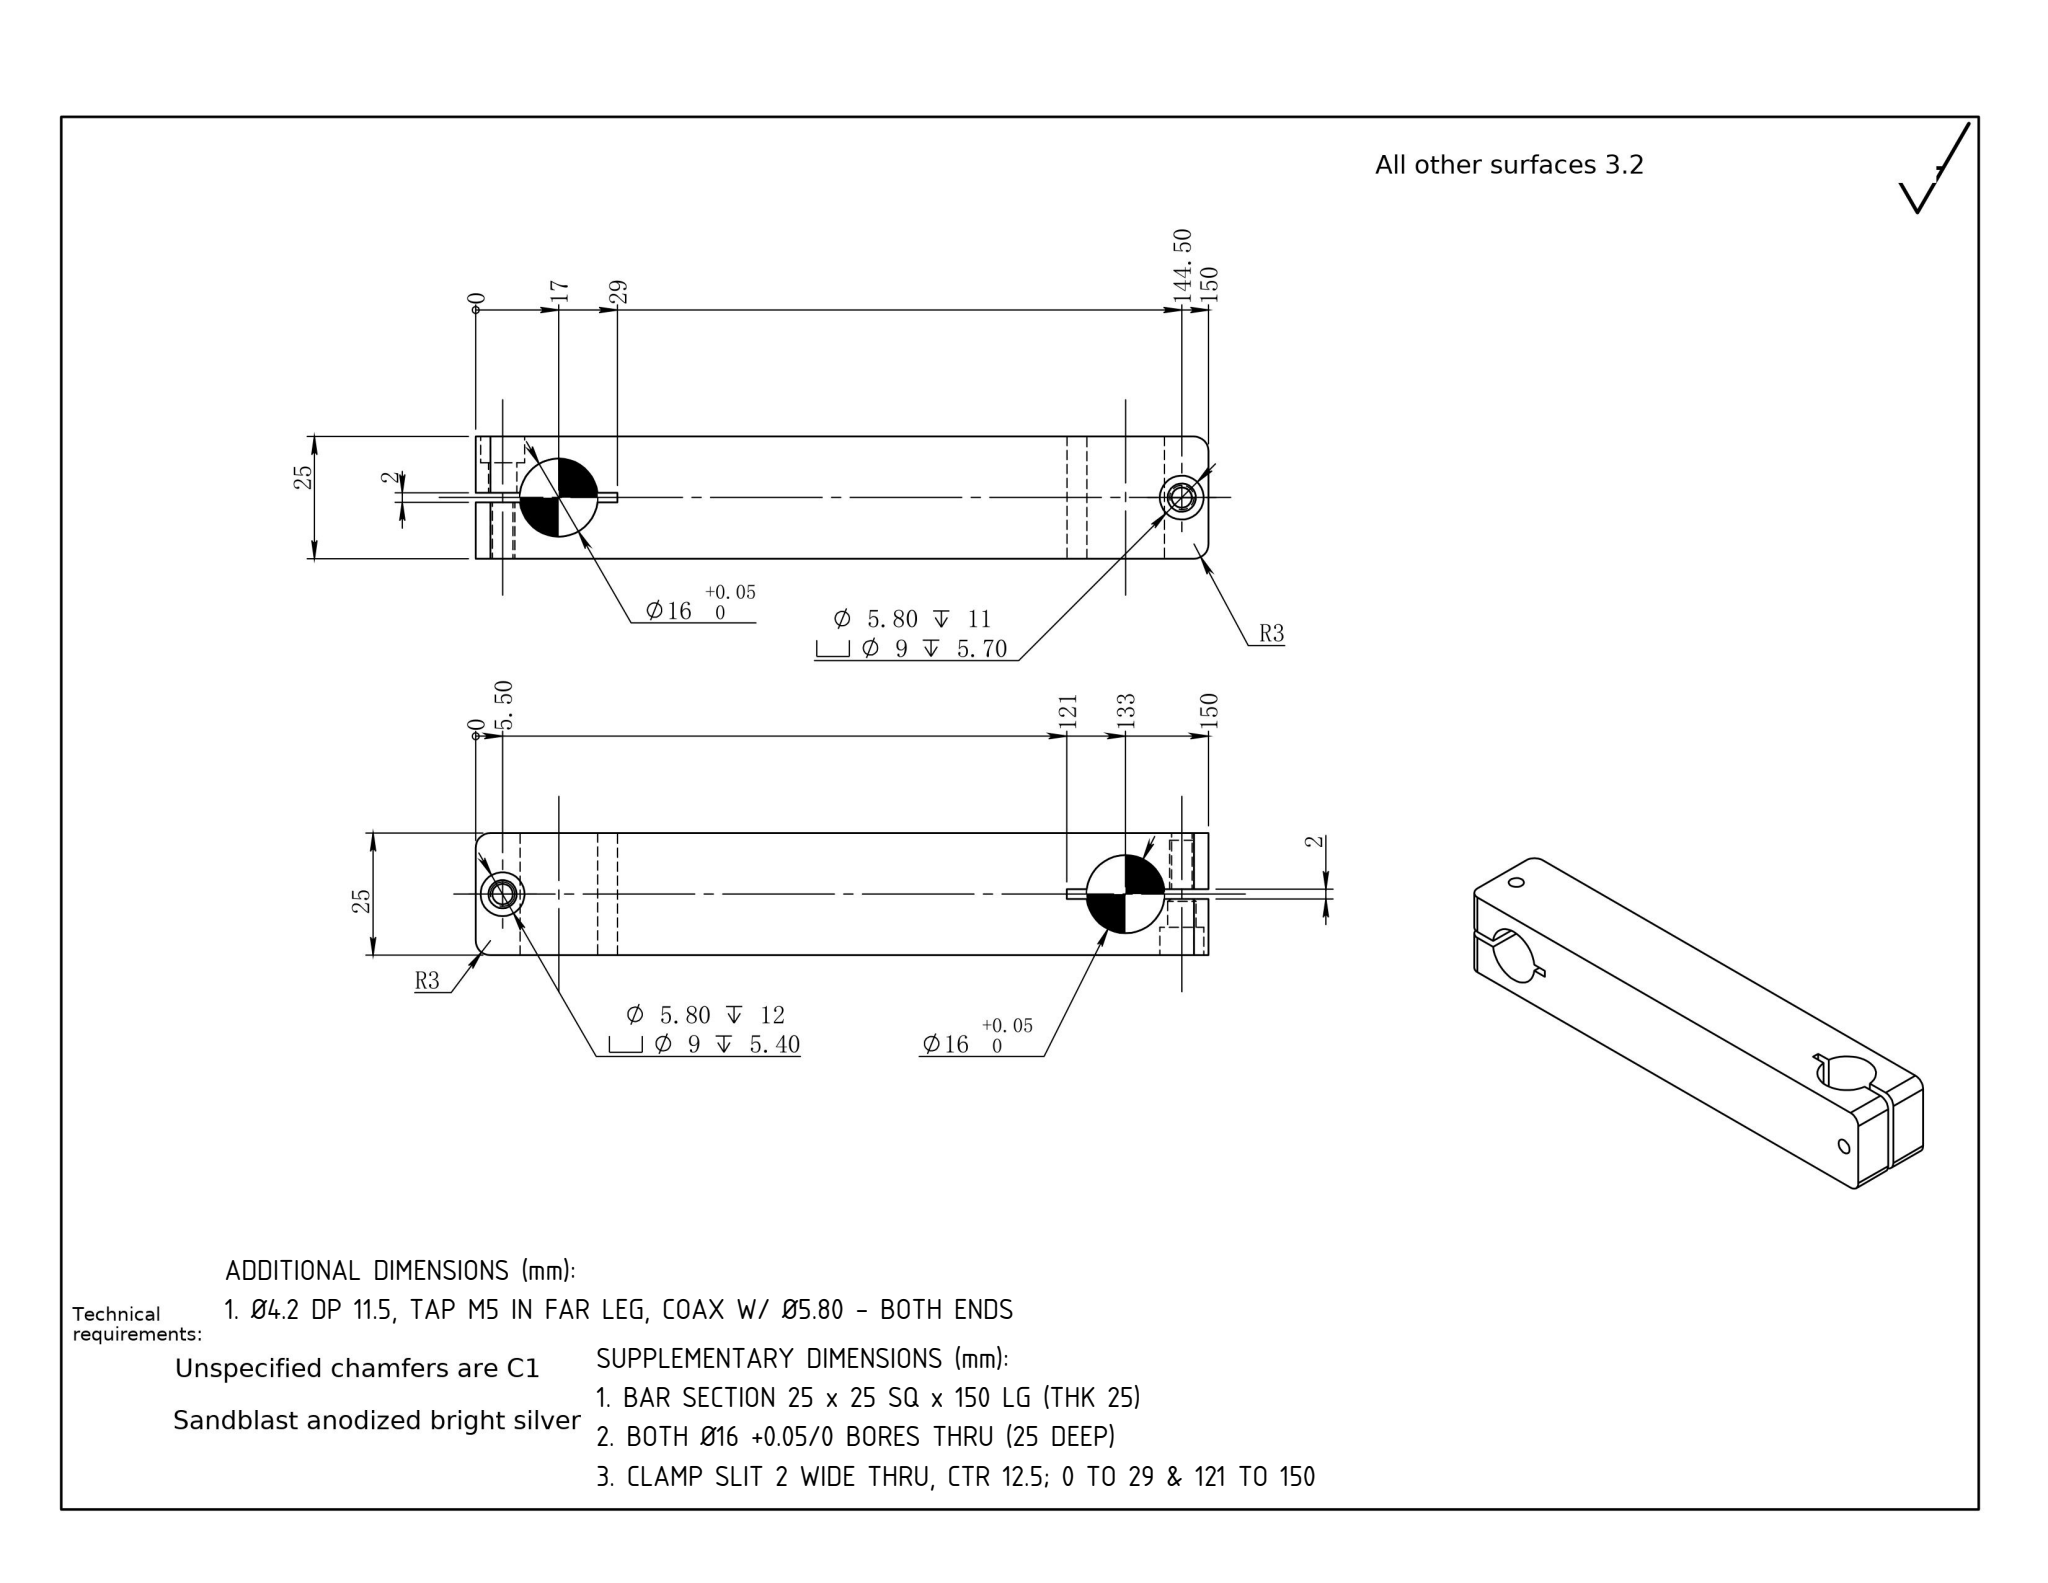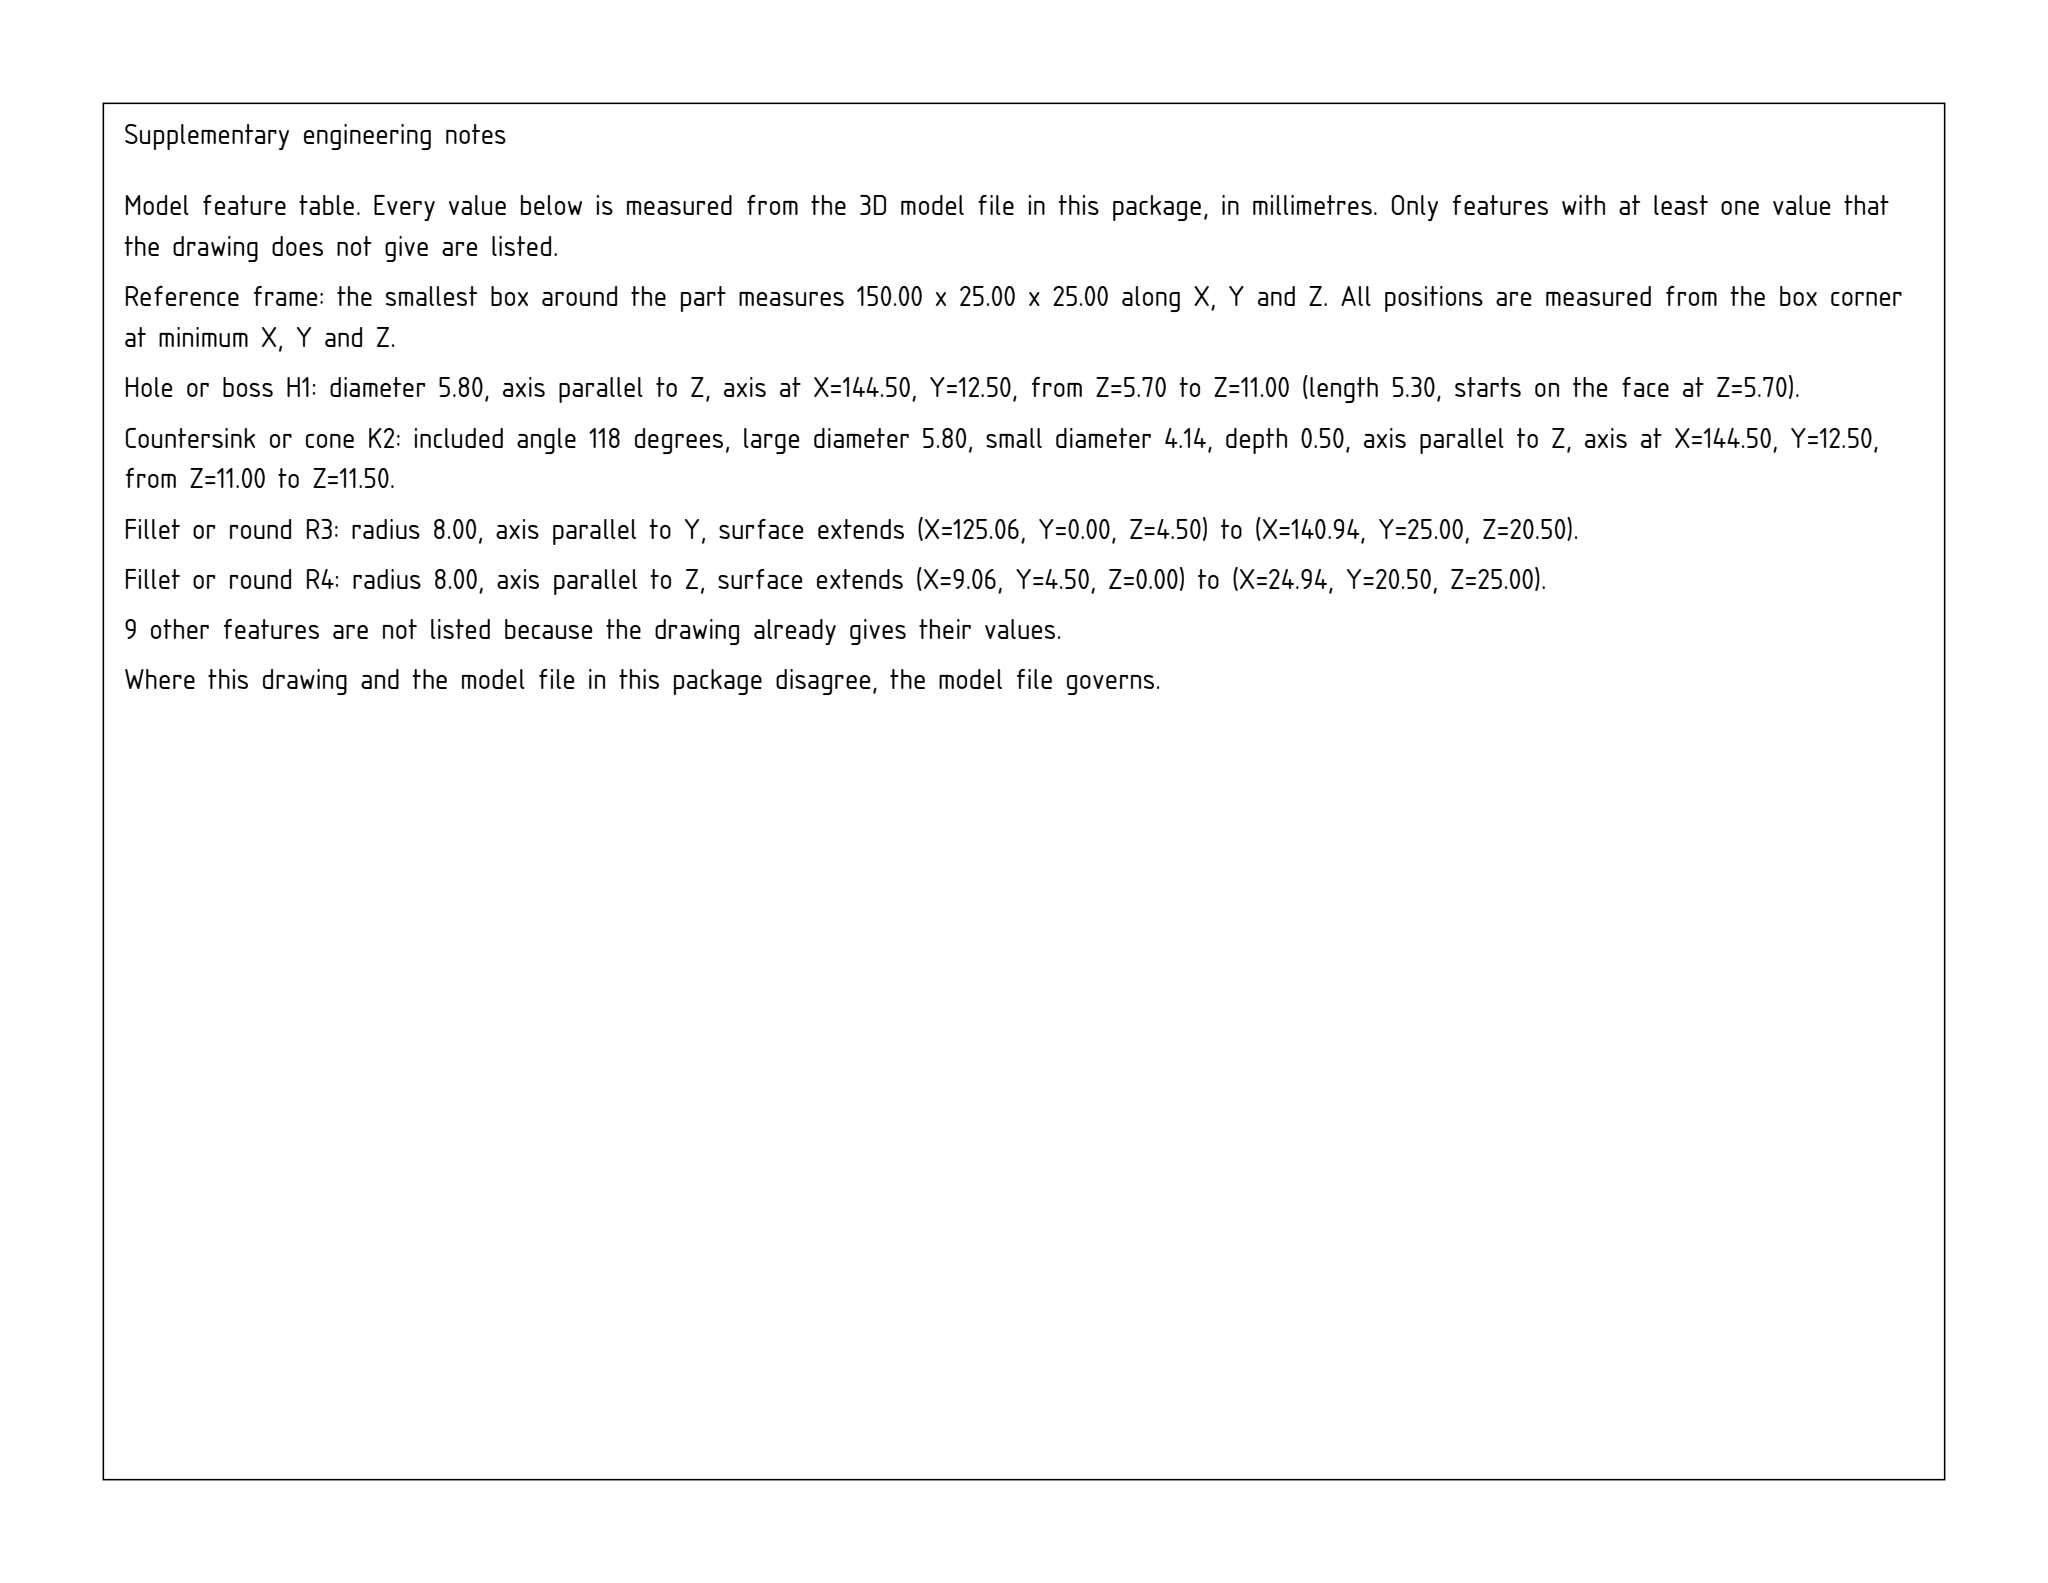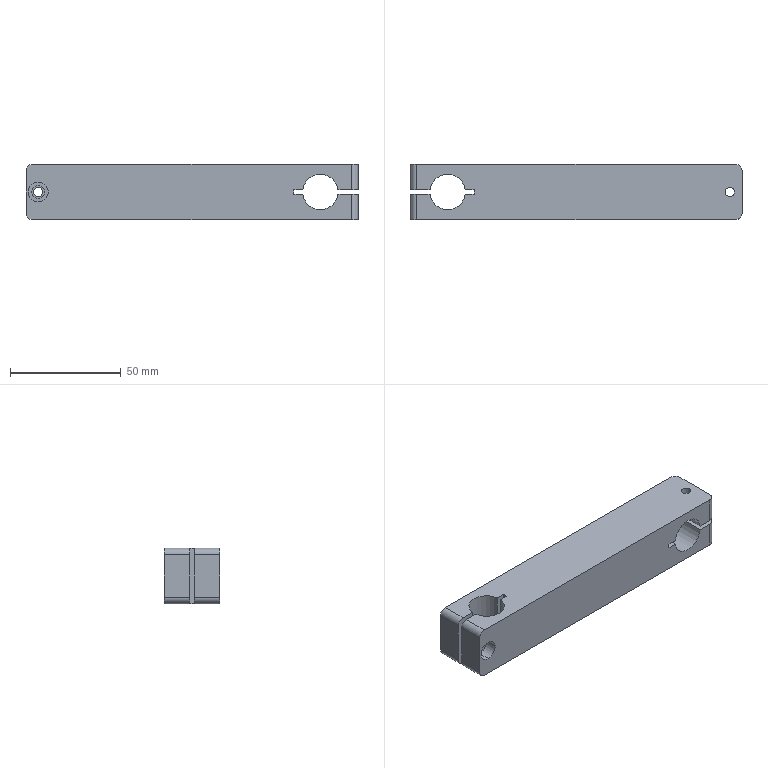Part | SolidWorks | mm | 1 solid | 47 faces | box 150 x 25 x 25 mm | volume 80879 mm3 | cylinder 25 | plane 20 | cone 2 | commonest cylinder face diameters 6 x8 16 x5 4.2 x4 9 x4 5.8 x4
build123d program:
from build123d import *

# Parameters (mm, degrees)
SKETCH1_W                                            = 150
SKETCH1_H                                            = 25
BOSS_EXTRUDE1_DEPTH                                  = 12.5
SKETCH2_R                                            = 8
CUT_EXTRUDE1_DEPTH                                   = 81.039
SKETCH3_W                                            = 29
SKETCH3_H                                            = 2
CUT_EXTRUDE2_DEPTH                                   = 81.039
SKETCH4_R                                            = 8
CUT_EXTRUDE3_DEPTH                                   = 81.039
SKETCH5_W                                            = 29
SKETCH5_H                                            = 2
CUT_EXTRUDE4_DEPTH                                   = 81.039
M5_HEX_SOCKET_HEAD_CAP_SCREW_CBORE1_D                = 5.8
M5_HEX_SOCKET_HEAD_CAP_SCREW_CBORE1_DEPTH            = 12
M5_HEX_SOCKET_HEAD_CAP_SCREW_CBORE1_CBORE_D          = 9
M5_HEX_SOCKET_HEAD_CAP_SCREW_CBORE1_CBORE_DEPTH      = 5.4
M5_HEX_SOCKET_HEAD_CAP_SCREW_CBORE1_TIP              = 1.742
HOLE_SIZE_ACCORDING_TO_THE_TYPE_OF_HEX_S_D           = 5.8
HOLE_SIZE_ACCORDING_TO_THE_TYPE_OF_HEX_S_DEPTH       = 11
HOLE_SIZE_ACCORDING_TO_THE_TYPE_OF_HEX_S_CBORE_D     = 9
HOLE_SIZE_ACCORDING_TO_THE_TYPE_OF_HEX_S_CBORE_DEPTH = 5.7
HOLE_SIZE_ACCORDING_TO_THE_TYPE_OF_HEX_S_TIP         = 1.742
M5_TAPPED_HOLE2_D                                    = 4.2
FILLET1_R                                            = 3


with BuildPart() as part:
    # Sketch1 → Boss-Extrude1 (new, symmetric)
    with BuildSketch(Plane.XY):
        Rectangle(SKETCH1_W, SKETCH1_H)
    extrude(amount=BOSS_EXTRUDE1_DEPTH, both=True)

    # Sketch2 → Cut-Extrude1 (cut, through all)
    with BuildSketch(Plane(origin=(0, 12.5, 0), x_dir=(1, 0, 0), z_dir=(0, 1, 0))):
        with Locations(Location((58, 0, 0), (0, 0, 270))):
            Circle(SKETCH2_R)
    extrude(amount=-CUT_EXTRUDE1_DEPTH, mode=Mode.SUBTRACT)

    # Sketch3 → Cut-Extrude2 (cut, through all)
    with BuildSketch(Plane(origin=(0, 12.5, 0), x_dir=(1, 0, 0), z_dir=(0, 1, 0))):
        with Locations((60.5, 0)):
            Rectangle(SKETCH3_W, SKETCH3_H)
    extrude(amount=-CUT_EXTRUDE2_DEPTH, mode=Mode.SUBTRACT)

    # Sketch4 → Cut-Extrude3 (cut, through all)
    with BuildSketch(Plane.XY.offset(12.5)):
        with Locations((-58, 0)):
            Circle(SKETCH4_R)
    extrude(amount=-CUT_EXTRUDE3_DEPTH, mode=Mode.SUBTRACT)

    # Sketch5 → Cut-Extrude4 (cut, through all)
    with BuildSketch(Plane.XY.offset(12.5)):
        with Locations((-60.5, 0)):
            Rectangle(SKETCH5_W, SKETCH5_H)
    extrude(amount=-CUT_EXTRUDE4_DEPTH, mode=Mode.SUBTRACT)

    # M5 Hex Socket Head Cap Screw CBORE1
    with Locations(Plane.XZ.offset(12.5)):
        with Locations((-69.5, 0)):
            CounterBoreHole(M5_HEX_SOCKET_HEAD_CAP_SCREW_CBORE1_D / 2, M5_HEX_SOCKET_HEAD_CAP_SCREW_CBORE1_CBORE_D / 2, M5_HEX_SOCKET_HEAD_CAP_SCREW_CBORE1_CBORE_DEPTH, depth=M5_HEX_SOCKET_HEAD_CAP_SCREW_CBORE1_DEPTH)
            with Locations((0, 0, -(M5_HEX_SOCKET_HEAD_CAP_SCREW_CBORE1_DEPTH + M5_HEX_SOCKET_HEAD_CAP_SCREW_CBORE1_TIP / 2))):  # 118° drill point
                Cone(0, M5_HEX_SOCKET_HEAD_CAP_SCREW_CBORE1_D / 2, M5_HEX_SOCKET_HEAD_CAP_SCREW_CBORE1_TIP, mode=Mode.SUBTRACT)

    # Hole Size according to the type of hex s
    with Locations(Plane(origin=(0, 0, -12.5), x_dir=(-1, 0, 0), z_dir=(0, 0, -1))):
        with Locations((-69.5, 0)):
            CounterBoreHole(HOLE_SIZE_ACCORDING_TO_THE_TYPE_OF_HEX_S_D / 2, HOLE_SIZE_ACCORDING_TO_THE_TYPE_OF_HEX_S_CBORE_D / 2, HOLE_SIZE_ACCORDING_TO_THE_TYPE_OF_HEX_S_CBORE_DEPTH, depth=HOLE_SIZE_ACCORDING_TO_THE_TYPE_OF_HEX_S_DEPTH)
            with Locations((0, 0, -(HOLE_SIZE_ACCORDING_TO_THE_TYPE_OF_HEX_S_DEPTH + HOLE_SIZE_ACCORDING_TO_THE_TYPE_OF_HEX_S_TIP / 2))):  # 118° drill point
                Cone(0, HOLE_SIZE_ACCORDING_TO_THE_TYPE_OF_HEX_S_D / 2, HOLE_SIZE_ACCORDING_TO_THE_TYPE_OF_HEX_S_TIP, mode=Mode.SUBTRACT)

    # M5 Tapped Hole2 (through all)
    with Locations(Plane.XZ.offset(-1)):
        with Locations((-69.5, 0)):
            Hole(M5_TAPPED_HOLE2_D / 2)

    # Sketch14 → M5 Tapped Hole1 (revolve, cut)
    with BuildSketch(Plane(origin=(69.5, 0, 1), x_dir=(0, 1, 0), z_dir=(1, 0, 0))):
        Polygon((0, 0), (0, 15.262), (2.1, 14), (2.1, 0), align=None)
    revolve(axis=Axis((69.5, 0, -5.35), (0, 0, 1)), mode=Mode.SUBTRACT)

    # Fillet1
    fillet1_edges = [part.edges().sort_by_distance(p)[0] for p in [
        (-75, 6.75, 12.5),
        (75, -12.5, -6.75),
        (75, 12.5, -6.75),
        (-75, 6.75, -12.5),
        (-75, -6.75, -12.5),
        (-75, -6.75, 12.5),
        (75, -12.5, 6.75),
        (75, 12.5, 6.75),
    ]]
    fillet(fillet1_edges, radius=FILLET1_R)


solid = part.part